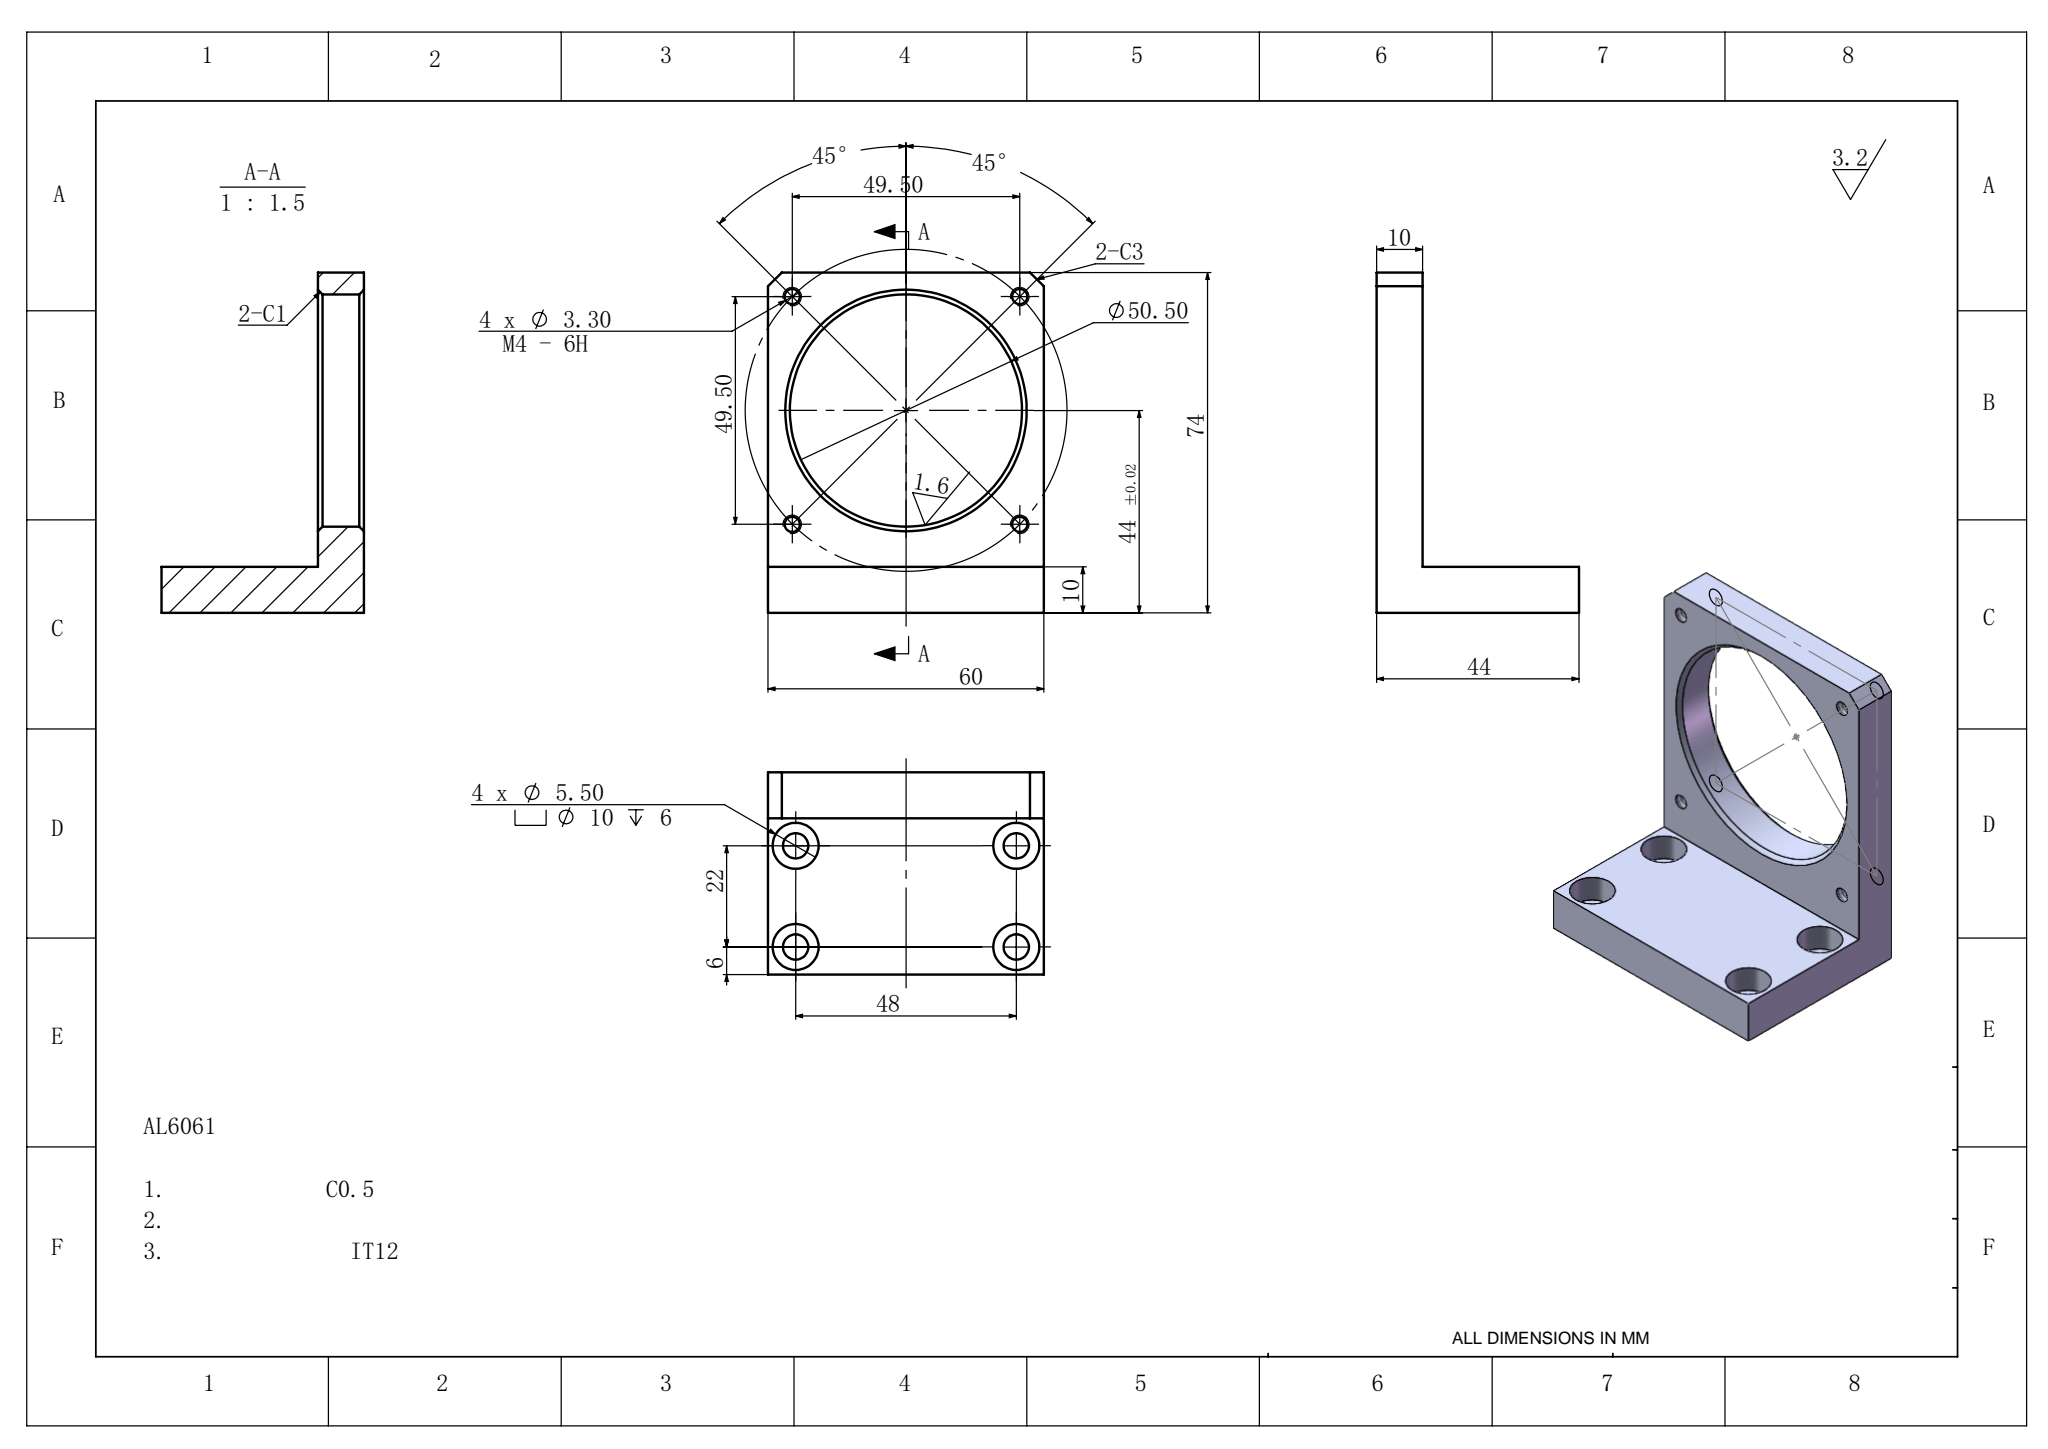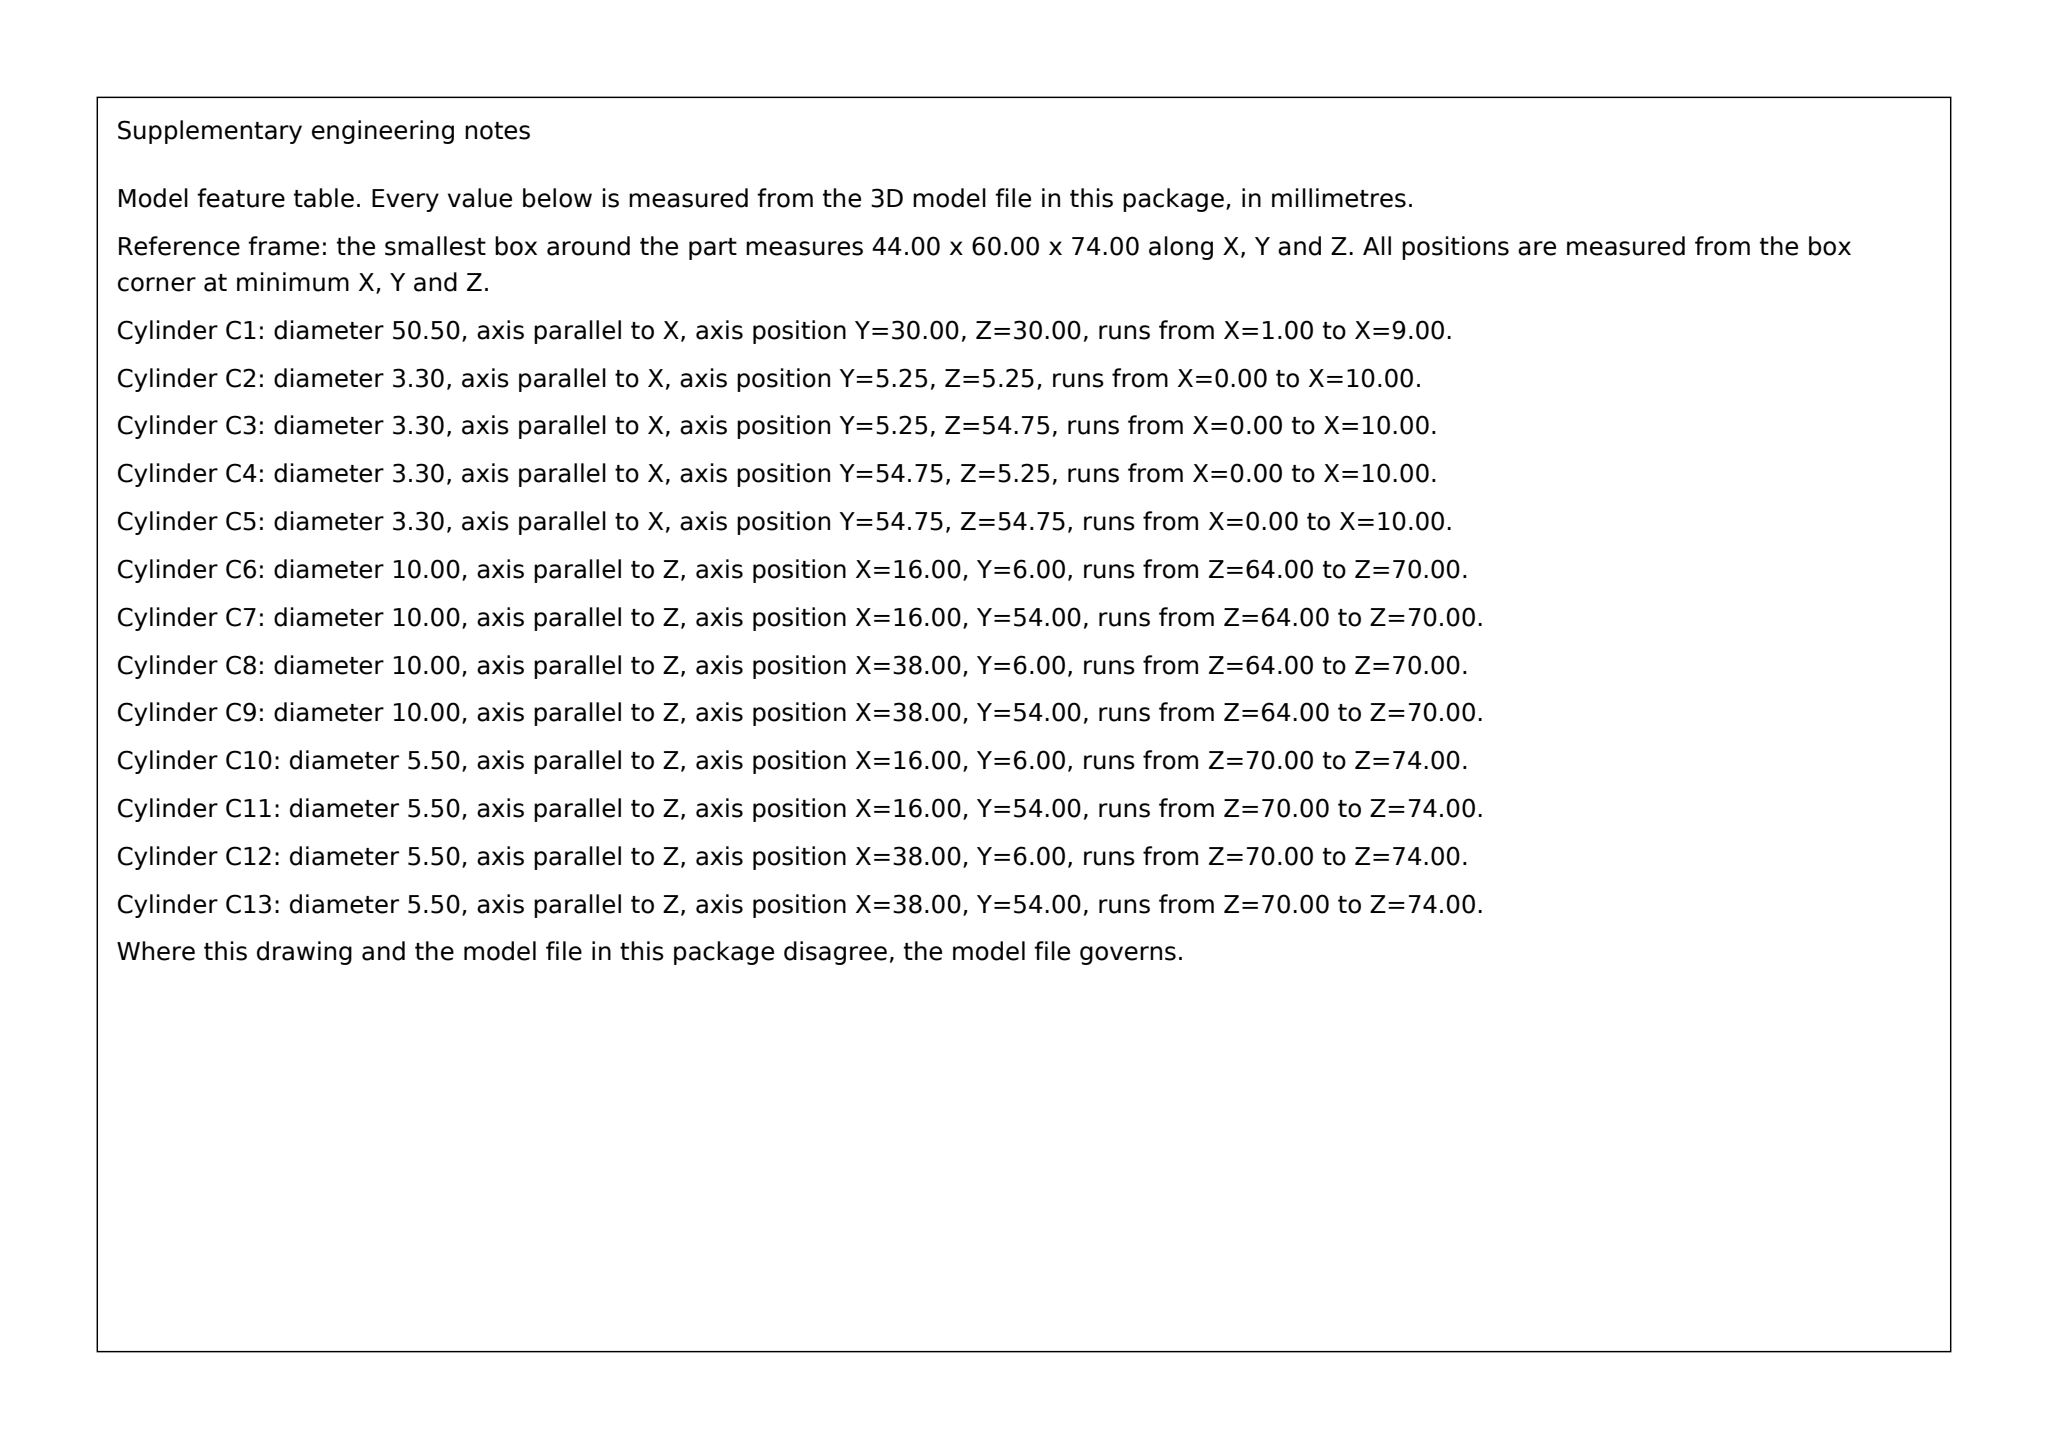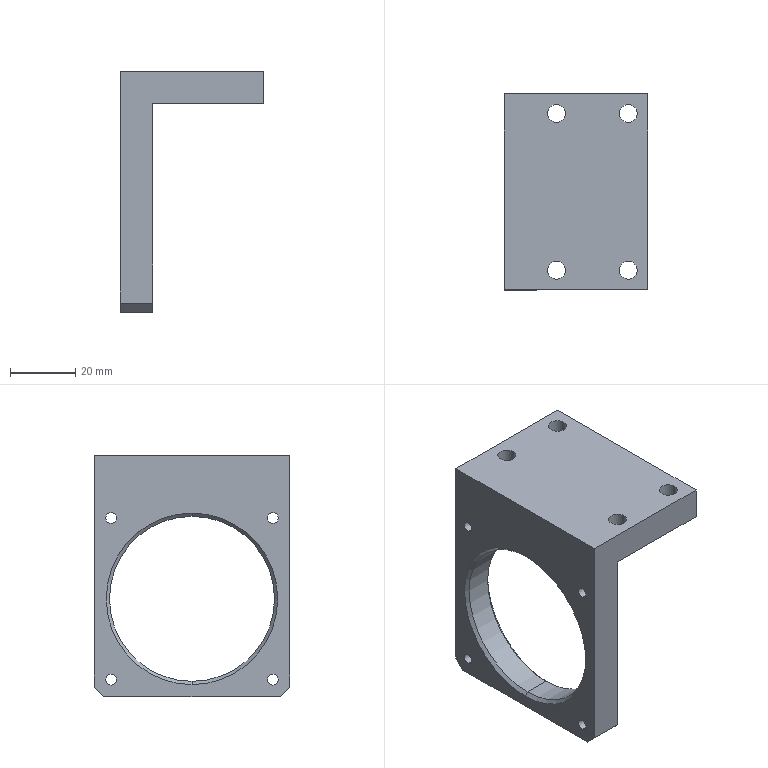Part | SolidWorks | mm | material AL6061 | 1 solid | 44 faces | box 44 x 60 x 74 mm | volume 41912 mm3 | cylinder 26 | plane 14 | cone 4 | commonest cylinder face diameters 3.3 x8 10 x8 5.5 x8 50.5 x2
build123d program:
from build123d import *

# Parameters (mm, degrees)
EXTRUDE1_DEPTH                                       = 60
SKETCH2_R                                            = 25.25
CUT_EXTRUDE1_DEPTH                                   = 10
CHAMFER1_SIZE                                        = 3
HOLE_SIZE_ACCORDING_TO_HEXAGON_SOCKET_HE_D           = 5.5
HOLE_SIZE_ACCORDING_TO_HEXAGON_SOCKET_HE_CBORE_D     = 10
HOLE_SIZE_ACCORDING_TO_HEXAGON_SOCKET_HE_CBORE_DEPTH = 6
M4_TAPPED_HOLE1_D                                    = 3.3
CHAMFER2_SIZE                                        = 1
CHAMFER3_SIZE                                        = 1


with BuildPart() as part:
    # Sketch1 → Extrude1 (new body)
    with BuildSketch(Plane(origin=(0, 0, 0), x_dir=(1, 0, 0), z_dir=(0, 1, 0))):
        Polygon((-48.691, 66.828), (-48.691, -7.172), (-4.691, -7.172), (-4.691, 2.828), (-38.691, 2.828), (-38.691, 66.828), align=None)
    extrude(amount=EXTRUDE1_DEPTH)

    # Sketch2 → Cut-Extrude1 (cut)
    with BuildSketch(Plane(origin=(-38.691, 0, 0), x_dir=(0, 0, -1), z_dir=(1, 0, 0))):
        with Locations((36.828, 30)):
            Circle(SKETCH2_R)
    extrude(amount=-CUT_EXTRUDE1_DEPTH, mode=Mode.SUBTRACT)

    # Chamfer1
    chamfer1_edges = [part.edges().sort_by_distance(p)[0] for p in [
        (-43.691, 60, -66.828),
        (-43.691, 0, -66.828),
    ]]
    chamfer(chamfer1_edges, length=CHAMFER1_SIZE)

    # Hole Size according to Hexagon Socket He (through all)
    with Locations(Plane(origin=(-10.691, 54, -2.828), x_dir=(-1, 0, 0), z_dir=(0, 0, -1))):
        with Locations((0, 0), (22, 0), (0, -48), (22, -48)):
            CounterBoreHole(HOLE_SIZE_ACCORDING_TO_HEXAGON_SOCKET_HE_D / 2, HOLE_SIZE_ACCORDING_TO_HEXAGON_SOCKET_HE_CBORE_D / 2, HOLE_SIZE_ACCORDING_TO_HEXAGON_SOCKET_HE_CBORE_DEPTH)

    # M4 Tapped Hole1 (through all)
    with Locations(Plane.ZY.offset(48.691)):
        with Locations((-61.578, 5.25), (-61.578, 54.75), (-12.078, 54.75), (-12.078, 5.25)):
            Hole(M4_TAPPED_HOLE1_D / 2)

    # Chamfer2
    chamfer2_edges = [part.edges().sort_by_distance(p)[0] for p in [
        (-48.691, 30, -11.578),
    ]]
    chamfer(chamfer2_edges, length=CHAMFER2_SIZE)

    # Chamfer3
    chamfer3_edges = [part.edges().sort_by_distance(p)[0] for p in [
        (-38.691, 30, -11.578),
    ]]
    chamfer(chamfer3_edges, length=CHAMFER3_SIZE)


solid = part.part